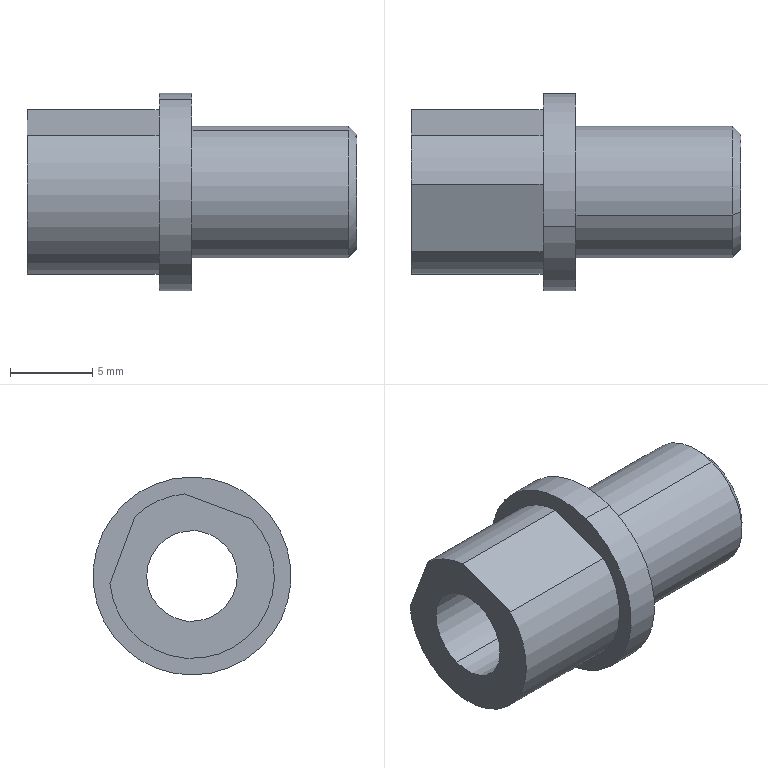Component | SolidWorks | 017NailOutlet-1 | 1 solid | 16 faces | box 20 x 12 x 12 mm | volume 856 mm3 | cylinder 8 | plane 6 | cone 2 | commonest cylinder face diameters 5.5 x2 8 x2 12 x2 10 x2
STEP:
#1=COLOUR_RGB('',0.7922,0.8196,0.9333);
#2=FILL_AREA_STYLE_COLOUR('',#1);
#3=FILL_AREA_STYLE('',(#2));
#4=SURFACE_STYLE_FILL_AREA(#3);
#5=SURFACE_SIDE_STYLE('',(#4));
#6=SURFACE_STYLE_USAGE(.BOTH.,#5);
#7=PRESENTATION_STYLE_ASSIGNMENT((#6));
#8=CARTESIAN_POINT('',(3.888,2.988,0.304));
#9=VERTEX_POINT('',#8);
#10=CARTESIAN_POINT('',(3.888,2.892,0.5621));
#11=VERTEX_POINT('',#10);
#12=CARTESIAN_POINT('',(3.888,2.94,0.4331));
#13=DIRECTION('',(1.,0.,0.));
#14=DIRECTION('',(0.,0.3505,-0.9366));
#15=AXIS2_PLACEMENT_3D('',#12,#13,#14);
#16=CIRCLE('',#15,0.1378);
#17=EDGE_CURVE('',#9,#11,#16,.T.);
#18=ORIENTED_EDGE('',*,*,#17,.F.);
#19=CARTESIAN_POINT('',(3.868,2.995,0.2856));
#20=VERTEX_POINT('',#19);
#21=CARTESIAN_POINT('',(3.888,2.988,0.304));
#22=DIRECTION('',(-0.7071,0.2478,-0.6623));
#23=VECTOR('',#22,39.37);
#24=LINE('',#21,#23);
#25=EDGE_CURVE('',#9,#20,#24,.T.);
#26=ORIENTED_EDGE('',*,*,#25,.T.);
#27=CARTESIAN_POINT('',(3.868,2.885,0.5806));
#28=VERTEX_POINT('',#27);
#29=CARTESIAN_POINT('',(3.868,2.94,0.4331));
#30=DIRECTION('',(-1.,-0.,-0.));
#31=DIRECTION('',(0.,0.3505,-0.9366));
#32=AXIS2_PLACEMENT_3D('',#29,#30,#31);
#33=CIRCLE('',#32,0.1575);
#34=EDGE_CURVE('',#28,#20,#33,.T.);
#35=ORIENTED_EDGE('',*,*,#34,.F.);
#36=CARTESIAN_POINT('',(3.888,2.892,0.5621));
#37=DIRECTION('',(-0.7071,-0.2478,0.6623));
#38=VECTOR('',#37,39.37);
#39=LINE('',#36,#38);
#40=EDGE_CURVE('',#11,#28,#39,.T.);
#41=ORIENTED_EDGE('',*,*,#40,.F.);
#42=EDGE_LOOP('',(#18,#26,#35,#41));
#43=FACE_OUTER_BOUND('',#42,.T.);
#44=CARTESIAN_POINT('',(3.888,2.94,0.4331));
#45=DIRECTION('',(-1.,-0.,-0.));
#46=DIRECTION('',(0.,-0.3505,0.9366));
#47=AXIS2_PLACEMENT_3D('',#44,#45,#46);
#48=CONICAL_SURFACE('',#47,0.1378,0.7854);
#49=ADVANCED_FACE('',(#43),#48,.T.);
#50=CARTESIAN_POINT('',(3.101,2.902,0.5345));
#51=VERTEX_POINT('',#50);
#52=CARTESIAN_POINT('',(3.101,2.978,0.3317));
#53=VERTEX_POINT('',#52);
#54=CARTESIAN_POINT('',(3.101,2.94,0.4331));
#55=DIRECTION('',(1.,0.,0.));
#56=DIRECTION('',(0.,0.3505,-0.9366));
#57=AXIS2_PLACEMENT_3D('',#54,#55,#56);
#58=CIRCLE('',#57,0.1083);
#59=EDGE_CURVE('',#51,#53,#58,.T.);
#60=ORIENTED_EDGE('',*,*,#59,.F.);
#61=CARTESIAN_POINT('',(3.888,2.902,0.5345));
#62=VERTEX_POINT('',#61);
#63=CARTESIAN_POINT('',(3.101,2.902,0.5345));
#64=DIRECTION('',(1.,0.,0.));
#65=VECTOR('',#64,39.37);
#66=LINE('',#63,#65);
#67=EDGE_CURVE('',#51,#62,#66,.T.);
#68=ORIENTED_EDGE('',*,*,#67,.T.);
#69=CARTESIAN_POINT('',(3.888,2.978,0.3317));
#70=VERTEX_POINT('',#69);
#71=CARTESIAN_POINT('',(3.888,2.94,0.4331));
#72=DIRECTION('',(1.,0.,0.));
#73=DIRECTION('',(0.,0.3505,-0.9366));
#74=AXIS2_PLACEMENT_3D('',#71,#72,#73);
#75=CIRCLE('',#74,0.1083);
#76=EDGE_CURVE('',#62,#70,#75,.T.);
#77=ORIENTED_EDGE('',*,*,#76,.T.);
#78=CARTESIAN_POINT('',(3.101,2.978,0.3317));
#79=DIRECTION('',(1.,0.,0.));
#80=VECTOR('',#79,39.37);
#81=LINE('',#78,#80);
#82=EDGE_CURVE('',#53,#70,#81,.T.);
#83=ORIENTED_EDGE('',*,*,#82,.F.);
#84=EDGE_LOOP('',(#60,#68,#77,#83));
#85=FACE_OUTER_BOUND('',#84,.T.);
#86=CARTESIAN_POINT('',(3.101,2.94,0.4331));
#87=DIRECTION('',(1.,0.,0.));
#88=DIRECTION('',(0.,0.3505,-0.9366));
#89=AXIS2_PLACEMENT_3D('',#86,#87,#88);
#90=CYLINDRICAL_SURFACE('',#89,0.1083);
#91=ADVANCED_FACE('',(#85),#90,.F.);
#92=ORIENTED_EDGE('',*,*,#34,.T.);
#93=CARTESIAN_POINT('',(3.494,2.995,0.2856));
#94=VERTEX_POINT('',#93);
#95=CARTESIAN_POINT('',(3.888,2.995,0.2856));
#96=DIRECTION('',(-1.,-0.,-0.));
#97=VECTOR('',#96,39.37);
#98=LINE('',#95,#97);
#99=EDGE_CURVE('',#20,#94,#98,.T.);
#100=ORIENTED_EDGE('',*,*,#99,.T.);
#101=CARTESIAN_POINT('',(3.494,2.885,0.5806));
#102=VERTEX_POINT('',#101);
#103=CARTESIAN_POINT('',(3.494,2.94,0.4331));
#104=DIRECTION('',(1.,0.,0.));
#105=DIRECTION('',(0.,0.3505,-0.9366));
#106=AXIS2_PLACEMENT_3D('',#103,#104,#105);
#107=CIRCLE('',#106,0.1575);
#108=EDGE_CURVE('',#94,#102,#107,.T.);
#109=ORIENTED_EDGE('',*,*,#108,.T.);
#110=CARTESIAN_POINT('',(3.888,2.885,0.5806));
#111=DIRECTION('',(-1.,-0.,-0.));
#112=VECTOR('',#111,39.37);
#113=LINE('',#110,#112);
#114=EDGE_CURVE('',#28,#102,#113,.T.);
#115=ORIENTED_EDGE('',*,*,#114,.F.);
#116=EDGE_LOOP('',(#92,#100,#109,#115));
#117=FACE_OUTER_BOUND('',#116,.T.);
#118=CARTESIAN_POINT('',(3.888,2.94,0.4331));
#119=DIRECTION('',(-1.,-0.,-0.));
#120=DIRECTION('',(0.,-0.3505,0.9366));
#121=AXIS2_PLACEMENT_3D('',#118,#119,#120);
#122=CYLINDRICAL_SURFACE('',#121,0.1575);
#123=ADVANCED_FACE('',(#117),#122,.T.);
#124=CARTESIAN_POINT('',(3.494,3.023,0.2118));
#125=VERTEX_POINT('',#124);
#126=CARTESIAN_POINT('',(3.494,2.857,0.6543));
#127=VERTEX_POINT('',#126);
#128=CARTESIAN_POINT('',(3.494,2.94,0.4331));
#129=DIRECTION('',(1.,0.,0.));
#130=DIRECTION('',(0.,0.3505,-0.9366));
#131=AXIS2_PLACEMENT_3D('',#128,#129,#130);
#132=CIRCLE('',#131,0.2362);
#133=EDGE_CURVE('',#125,#127,#132,.T.);
#134=ORIENTED_EDGE('',*,*,#133,.F.);
#135=CARTESIAN_POINT('',(3.416,3.023,0.2118));
#136=VERTEX_POINT('',#135);
#137=CARTESIAN_POINT('',(3.494,3.023,0.2118));
#138=DIRECTION('',(-1.,-0.,-0.));
#139=VECTOR('',#138,39.37);
#140=LINE('',#137,#139);
#141=EDGE_CURVE('',#125,#136,#140,.T.);
#142=ORIENTED_EDGE('',*,*,#141,.T.);
#143=CARTESIAN_POINT('',(3.416,2.857,0.6543));
#144=VERTEX_POINT('',#143);
#145=CARTESIAN_POINT('',(3.416,2.94,0.4331));
#146=DIRECTION('',(1.,0.,0.));
#147=DIRECTION('',(0.,0.3505,-0.9366));
#148=AXIS2_PLACEMENT_3D('',#145,#146,#147);
#149=CIRCLE('',#148,0.2362);
#150=EDGE_CURVE('',#136,#144,#149,.T.);
#151=ORIENTED_EDGE('',*,*,#150,.T.);
#152=CARTESIAN_POINT('',(3.494,2.857,0.6543));
#153=DIRECTION('',(-1.,-0.,-0.));
#154=VECTOR('',#153,39.37);
#155=LINE('',#152,#154);
#156=EDGE_CURVE('',#127,#144,#155,.T.);
#157=ORIENTED_EDGE('',*,*,#156,.F.);
#158=EDGE_LOOP('',(#134,#142,#151,#157));
#159=FACE_OUTER_BOUND('',#158,.T.);
#160=CARTESIAN_POINT('',(3.494,2.94,0.4331));
#161=DIRECTION('',(-1.,-0.,-0.));
#162=DIRECTION('',(0.,-0.3505,0.9366));
#163=AXIS2_PLACEMENT_3D('',#160,#161,#162);
#164=CYLINDRICAL_SURFACE('',#163,0.2362);
#165=ADVANCED_FACE('',(#159),#164,.T.);
#166=CARTESIAN_POINT('',(3.416,3.076,0.5755));
#167=VERTEX_POINT('',#166);
#168=CARTESIAN_POINT('',(3.416,2.958,0.6291));
#169=VERTEX_POINT('',#168);
#170=CARTESIAN_POINT('',(3.416,2.94,0.4331));
#171=DIRECTION('',(1.,0.,0.));
#172=DIRECTION('',(0.,0.3505,-0.9366));
#173=AXIS2_PLACEMENT_3D('',#170,#171,#172);
#174=CIRCLE('',#173,0.1969);
#175=EDGE_CURVE('',#167,#169,#174,.T.);
#176=ORIENTED_EDGE('',*,*,#175,.F.);
#177=CARTESIAN_POINT('',(3.101,3.076,0.5755));
#178=VERTEX_POINT('',#177);
#179=CARTESIAN_POINT('',(3.416,3.076,0.5755));
#180=DIRECTION('',(-1.,-0.,-0.));
#181=VECTOR('',#180,39.37);
#182=LINE('',#179,#181);
#183=EDGE_CURVE('',#167,#178,#182,.T.);
#184=ORIENTED_EDGE('',*,*,#183,.T.);
#185=CARTESIAN_POINT('',(3.101,2.958,0.6291));
#186=VERTEX_POINT('',#185);
#187=CARTESIAN_POINT('',(3.101,2.94,0.4331));
#188=DIRECTION('',(1.,0.,0.));
#189=DIRECTION('',(0.,0.3505,-0.9366));
#190=AXIS2_PLACEMENT_3D('',#187,#188,#189);
#191=CIRCLE('',#190,0.1969);
#192=EDGE_CURVE('',#178,#186,#191,.T.);
#193=ORIENTED_EDGE('',*,*,#192,.T.);
#194=CARTESIAN_POINT('',(3.416,2.958,0.6291));
#195=DIRECTION('',(-1.,-0.,-0.));
#196=VECTOR('',#195,39.37);
#197=LINE('',#194,#196);
#198=EDGE_CURVE('',#169,#186,#197,.T.);
#199=ORIENTED_EDGE('',*,*,#198,.F.);
#200=EDGE_LOOP('',(#176,#184,#193,#199));
#201=FACE_OUTER_BOUND('',#200,.T.);
#202=CARTESIAN_POINT('',(3.416,2.94,0.4331));
#203=DIRECTION('',(-1.,-0.,-0.));
#204=DIRECTION('',(0.,-0.3505,0.9366));
#205=AXIS2_PLACEMENT_3D('',#202,#203,#204);
#206=CYLINDRICAL_SURFACE('',#205,0.1969);
#207=ADVANCED_FACE('',(#201),#206,.T.);
#208=CARTESIAN_POINT('',(3.494,2.94,0.4331));
#209=DIRECTION('',(1.,0.,0.));
#210=DIRECTION('',(0.,0.3505,-0.9366));
#211=AXIS2_PLACEMENT_3D('',#208,#209,#210);
#212=CIRCLE('',#211,0.2362);
#213=EDGE_CURVE('',#127,#125,#212,.T.);
#214=ORIENTED_EDGE('',*,*,#213,.T.);
#215=ORIENTED_EDGE('',*,*,#133,.T.);
#216=EDGE_LOOP('',(#214,#215));
#217=FACE_OUTER_BOUND('',#216,.T.);
#218=CARTESIAN_POINT('',(3.494,2.94,0.4331));
#219=DIRECTION('',(1.,0.,0.));
#220=DIRECTION('',(0.,0.3505,-0.9366));
#221=AXIS2_PLACEMENT_3D('',#218,#219,#220);
#222=CIRCLE('',#221,0.1575);
#223=EDGE_CURVE('',#102,#94,#222,.T.);
#224=ORIENTED_EDGE('',*,*,#223,.F.);
#225=ORIENTED_EDGE('',*,*,#108,.F.);
#226=EDGE_LOOP('',(#224,#225));
#227=FACE_BOUND('',#226,.T.);
#228=CARTESIAN_POINT('',(3.494,2.94,0.4331));
#229=DIRECTION('',(1.,0.,0.));
#230=DIRECTION('',(-0.,0.3505,-0.9366));
#231=AXIS2_PLACEMENT_3D('',#228,#229,#230);
#232=PLANE('',#231);
#233=ADVANCED_FACE('',(#217,#227),#232,.T.);
#234=CARTESIAN_POINT('',(3.101,2.798,0.5689));
#235=VERTEX_POINT('',#234);
#236=CARTESIAN_POINT('',(3.101,3.136,0.4148));
#237=VERTEX_POINT('',#236);
#238=CARTESIAN_POINT('',(3.101,2.94,0.4331));
#239=DIRECTION('',(1.,0.,0.));
#240=DIRECTION('',(0.,0.3505,-0.9366));
#241=AXIS2_PLACEMENT_3D('',#238,#239,#240);
#242=CIRCLE('',#241,0.1969);
#243=EDGE_CURVE('',#235,#237,#242,.T.);
#244=ORIENTED_EDGE('',*,*,#243,.T.);
#245=CARTESIAN_POINT('',(3.416,3.136,0.4148));
#246=VERTEX_POINT('',#245);
#247=CARTESIAN_POINT('',(3.416,3.136,0.4148));
#248=DIRECTION('',(-1.,-0.,-0.));
#249=VECTOR('',#248,39.37);
#250=LINE('',#247,#249);
#251=EDGE_CURVE('',#246,#237,#250,.T.);
#252=ORIENTED_EDGE('',*,*,#251,.F.);
#253=CARTESIAN_POINT('',(3.416,2.798,0.5689));
#254=VERTEX_POINT('',#253);
#255=CARTESIAN_POINT('',(3.416,2.94,0.4331));
#256=DIRECTION('',(1.,0.,0.));
#257=DIRECTION('',(0.,0.3505,-0.9366));
#258=AXIS2_PLACEMENT_3D('',#255,#256,#257);
#259=CIRCLE('',#258,0.1969);
#260=EDGE_CURVE('',#254,#246,#259,.T.);
#261=ORIENTED_EDGE('',*,*,#260,.F.);
#262=CARTESIAN_POINT('',(3.416,2.798,0.5689));
#263=DIRECTION('',(-1.,-0.,-0.));
#264=VECTOR('',#263,39.37);
#265=LINE('',#262,#264);
#266=EDGE_CURVE('',#254,#235,#265,.T.);
#267=ORIENTED_EDGE('',*,*,#266,.T.);
#268=EDGE_LOOP('',(#244,#252,#261,#267));
#269=FACE_OUTER_BOUND('',#268,.T.);
#270=CARTESIAN_POINT('',(3.416,2.94,0.4331));
#271=DIRECTION('',(-1.,-0.,-0.));
#272=DIRECTION('',(0.,-0.3505,0.9366));
#273=AXIS2_PLACEMENT_3D('',#270,#271,#272);
#274=CYLINDRICAL_SURFACE('',#273,0.1969);
#275=ADVANCED_FACE('',(#269),#274,.T.);
#276=CARTESIAN_POINT('',(3.101,2.94,0.4331));
#277=DIRECTION('',(1.,0.,0.));
#278=DIRECTION('',(0.,0.3505,-0.9366));
#279=AXIS2_PLACEMENT_3D('',#276,#277,#278);
#280=CIRCLE('',#279,0.1083);
#281=EDGE_CURVE('',#53,#51,#280,.T.);
#282=ORIENTED_EDGE('',*,*,#281,.T.);
#283=ORIENTED_EDGE('',*,*,#59,.T.);
#284=EDGE_LOOP('',(#282,#283));
#285=FACE_BOUND('',#284,.T.);
#286=ORIENTED_EDGE('',*,*,#192,.F.);
#287=CARTESIAN_POINT('',(3.101,3.136,0.4148));
#288=DIRECTION('',(0.,-0.3505,0.9366));
#289=VECTOR('',#288,39.37);
#290=LINE('',#287,#289);
#291=EDGE_CURVE('',#237,#178,#290,.T.);
#292=ORIENTED_EDGE('',*,*,#291,.F.);
#293=ORIENTED_EDGE('',*,*,#243,.F.);
#294=CARTESIAN_POINT('',(3.101,2.958,0.6291));
#295=DIRECTION('',(0.,-0.9366,-0.3505));
#296=VECTOR('',#295,39.37);
#297=LINE('',#294,#296);
#298=EDGE_CURVE('',#186,#235,#297,.T.);
#299=ORIENTED_EDGE('',*,*,#298,.F.);
#300=EDGE_LOOP('',(#286,#292,#293,#299));
#301=FACE_OUTER_BOUND('',#300,.T.);
#302=CARTESIAN_POINT('',(3.101,2.94,0.4331));
#303=DIRECTION('',(1.,0.,0.));
#304=DIRECTION('',(-0.,0.3505,-0.9366));
#305=AXIS2_PLACEMENT_3D('',#302,#303,#304);
#306=PLANE('',#305);
#307=ADVANCED_FACE('',(#285,#301),#306,.F.);
#308=CARTESIAN_POINT('',(3.416,2.94,0.4331));
#309=DIRECTION('',(1.,0.,0.));
#310=DIRECTION('',(0.,0.3505,-0.9366));
#311=AXIS2_PLACEMENT_3D('',#308,#309,#310);
#312=CIRCLE('',#311,0.2362);
#313=EDGE_CURVE('',#144,#136,#312,.T.);
#314=ORIENTED_EDGE('',*,*,#313,.F.);
#315=ORIENTED_EDGE('',*,*,#150,.F.);
#316=EDGE_LOOP('',(#314,#315));
#317=FACE_OUTER_BOUND('',#316,.T.);
#318=ORIENTED_EDGE('',*,*,#260,.T.);
#319=CARTESIAN_POINT('',(3.416,3.136,0.4148));
#320=DIRECTION('',(0.,-0.3505,0.9366));
#321=VECTOR('',#320,39.37);
#322=LINE('',#319,#321);
#323=EDGE_CURVE('',#246,#167,#322,.T.);
#324=ORIENTED_EDGE('',*,*,#323,.T.);
#325=ORIENTED_EDGE('',*,*,#175,.T.);
#326=CARTESIAN_POINT('',(3.416,2.958,0.6291));
#327=DIRECTION('',(0.,-0.9366,-0.3505));
#328=VECTOR('',#327,39.37);
#329=LINE('',#326,#328);
#330=EDGE_CURVE('',#169,#254,#329,.T.);
#331=ORIENTED_EDGE('',*,*,#330,.T.);
#332=EDGE_LOOP('',(#318,#324,#325,#331));
#333=FACE_BOUND('',#332,.T.);
#334=CARTESIAN_POINT('',(3.416,2.94,0.4331));
#335=DIRECTION('',(1.,0.,0.));
#336=DIRECTION('',(-0.,0.3505,-0.9366));
#337=AXIS2_PLACEMENT_3D('',#334,#335,#336);
#338=PLANE('',#337);
#339=ADVANCED_FACE('',(#317,#333),#338,.F.);
#340=ORIENTED_EDGE('',*,*,#141,.F.);
#341=ORIENTED_EDGE('',*,*,#213,.F.);
#342=ORIENTED_EDGE('',*,*,#156,.T.);
#343=ORIENTED_EDGE('',*,*,#313,.T.);
#344=EDGE_LOOP('',(#340,#341,#342,#343));
#345=FACE_OUTER_BOUND('',#344,.T.);
#346=CARTESIAN_POINT('',(3.494,2.94,0.4331));
#347=DIRECTION('',(-1.,-0.,-0.));
#348=DIRECTION('',(0.,-0.3505,0.9366));
#349=AXIS2_PLACEMENT_3D('',#346,#347,#348);
#350=CYLINDRICAL_SURFACE('',#349,0.2362);
#351=ADVANCED_FACE('',(#345),#350,.T.);
#352=ORIENTED_EDGE('',*,*,#99,.F.);
#353=CARTESIAN_POINT('',(3.868,2.94,0.4331));
#354=DIRECTION('',(-1.,-0.,-0.));
#355=DIRECTION('',(0.,0.3505,-0.9366));
#356=AXIS2_PLACEMENT_3D('',#353,#354,#355);
#357=CIRCLE('',#356,0.1575);
#358=EDGE_CURVE('',#20,#28,#357,.T.);
#359=ORIENTED_EDGE('',*,*,#358,.T.);
#360=ORIENTED_EDGE('',*,*,#114,.T.);
#361=ORIENTED_EDGE('',*,*,#223,.T.);
#362=EDGE_LOOP('',(#352,#359,#360,#361));
#363=FACE_OUTER_BOUND('',#362,.T.);
#364=CARTESIAN_POINT('',(3.888,2.94,0.4331));
#365=DIRECTION('',(-1.,-0.,-0.));
#366=DIRECTION('',(0.,-0.3505,0.9366));
#367=AXIS2_PLACEMENT_3D('',#364,#365,#366);
#368=CYLINDRICAL_SURFACE('',#367,0.1575);
#369=ADVANCED_FACE('',(#363),#368,.T.);
#370=CARTESIAN_POINT('',(3.888,2.94,0.4331));
#371=DIRECTION('',(1.,0.,0.));
#372=DIRECTION('',(0.,0.3505,-0.9366));
#373=AXIS2_PLACEMENT_3D('',#370,#371,#372);
#374=CIRCLE('',#373,0.1378);
#375=EDGE_CURVE('',#11,#9,#374,.T.);
#376=ORIENTED_EDGE('',*,*,#375,.T.);
#377=ORIENTED_EDGE('',*,*,#17,.T.);
#378=EDGE_LOOP('',(#376,#377));
#379=FACE_OUTER_BOUND('',#378,.T.);
#380=CARTESIAN_POINT('',(3.888,2.94,0.4331));
#381=DIRECTION('',(1.,0.,0.));
#382=DIRECTION('',(0.,0.3505,-0.9366));
#383=AXIS2_PLACEMENT_3D('',#380,#381,#382);
#384=CIRCLE('',#383,0.1083);
#385=EDGE_CURVE('',#70,#62,#384,.T.);
#386=ORIENTED_EDGE('',*,*,#385,.F.);
#387=ORIENTED_EDGE('',*,*,#76,.F.);
#388=EDGE_LOOP('',(#386,#387));
#389=FACE_BOUND('',#388,.T.);
#390=CARTESIAN_POINT('',(3.888,2.94,0.4331));
#391=DIRECTION('',(1.,0.,0.));
#392=DIRECTION('',(-0.,0.3505,-0.9366));
#393=AXIS2_PLACEMENT_3D('',#390,#391,#392);
#394=PLANE('',#393);
#395=ADVANCED_FACE('',(#379,#389),#394,.T.);
#396=ORIENTED_EDGE('',*,*,#67,.F.);
#397=ORIENTED_EDGE('',*,*,#281,.F.);
#398=ORIENTED_EDGE('',*,*,#82,.T.);
#399=ORIENTED_EDGE('',*,*,#385,.T.);
#400=EDGE_LOOP('',(#396,#397,#398,#399));
#401=FACE_OUTER_BOUND('',#400,.T.);
#402=CARTESIAN_POINT('',(3.101,2.94,0.4331));
#403=DIRECTION('',(1.,0.,0.));
#404=DIRECTION('',(0.,0.3505,-0.9366));
#405=AXIS2_PLACEMENT_3D('',#402,#403,#404);
#406=CYLINDRICAL_SURFACE('',#405,0.1083);
#407=ADVANCED_FACE('',(#401),#406,.F.);
#408=ORIENTED_EDGE('',*,*,#25,.F.);
#409=ORIENTED_EDGE('',*,*,#375,.F.);
#410=ORIENTED_EDGE('',*,*,#40,.T.);
#411=ORIENTED_EDGE('',*,*,#358,.F.);
#412=EDGE_LOOP('',(#408,#409,#410,#411));
#413=FACE_OUTER_BOUND('',#412,.T.);
#414=CARTESIAN_POINT('',(3.888,2.94,0.4331));
#415=DIRECTION('',(-1.,-0.,-0.));
#416=DIRECTION('',(0.,-0.3505,0.9366));
#417=AXIS2_PLACEMENT_3D('',#414,#415,#416);
#418=CONICAL_SURFACE('',#417,0.1378,0.7854);
#419=ADVANCED_FACE('',(#413),#418,.T.);
#420=ORIENTED_EDGE('',*,*,#298,.T.);
#421=ORIENTED_EDGE('',*,*,#266,.F.);
#422=ORIENTED_EDGE('',*,*,#330,.F.);
#423=ORIENTED_EDGE('',*,*,#198,.T.);
#424=EDGE_LOOP('',(#420,#421,#422,#423));
#425=FACE_OUTER_BOUND('',#424,.T.);
#426=CARTESIAN_POINT('',(3.416,2.958,0.6291));
#427=DIRECTION('',(-0.,0.3505,-0.9366));
#428=DIRECTION('',(-1.,-0.,-0.));
#429=AXIS2_PLACEMENT_3D('',#426,#427,#428);
#430=PLANE('',#429);
#431=ADVANCED_FACE('',(#425),#430,.F.);
#432=ORIENTED_EDGE('',*,*,#291,.T.);
#433=ORIENTED_EDGE('',*,*,#183,.F.);
#434=ORIENTED_EDGE('',*,*,#323,.F.);
#435=ORIENTED_EDGE('',*,*,#251,.T.);
#436=EDGE_LOOP('',(#432,#433,#434,#435));
#437=FACE_OUTER_BOUND('',#436,.T.);
#438=CARTESIAN_POINT('',(3.416,3.136,0.4148));
#439=DIRECTION('',(0.,-0.9366,-0.3505));
#440=DIRECTION('',(-0.,0.3505,-0.9366));
#441=AXIS2_PLACEMENT_3D('',#438,#439,#440);
#442=PLANE('',#441);
#443=ADVANCED_FACE('',(#437),#442,.F.);
#444=CLOSED_SHELL('',(#49,#91,#123,#165,#207,#233,#275,#307,#339,#351,#369,#395,#407,#419,#431,#443));
#445=MANIFOLD_SOLID_BREP('',#444);
#446=STYLED_ITEM('',(#7),#445);
#447=PRESENTATION_LAYER_ASSIGNMENT('','',(#446));
#448=CARTESIAN_POINT('',(0.,0.,0.));
#449=DIRECTION('',(0.,0.,1.));
#450=DIRECTION('',(1.,0.,0.));
#451=AXIS2_PLACEMENT_3D('',#448,#449,#450);
#452=(LENGTH_UNIT()NAMED_UNIT(*)SI_UNIT($,.METRE.));
#453=LENGTH_MEASURE_WITH_UNIT(LENGTH_MEASURE(0.0254),#452);
#454=DIMENSIONAL_EXPONENTS(1.,0.,0.,0.,0.,0.,0.);
#455=(CONVERSION_BASED_UNIT('',#453)LENGTH_UNIT()NAMED_UNIT(#454));
#456=UNCERTAINTY_MEASURE_WITH_UNIT(LENGTH_MEASURE(0.00001),#455,'','');
#457=(NAMED_UNIT(*)PLANE_ANGLE_UNIT()SI_UNIT($,.RADIAN.));
#458=(NAMED_UNIT(*)SI_UNIT($,.STERADIAN.)SOLID_ANGLE_UNIT());
#459=(GEOMETRIC_REPRESENTATION_CONTEXT(3)GLOBAL_UNCERTAINTY_ASSIGNED_CONTEXT((#456))GLOBAL_UNIT_ASSIGNED_CONTEXT((#455,#457,#458))REPRESENTATION_CONTEXT('',''));
#460=ADVANCED_BREP_SHAPE_REPRESENTATION('',(#445,#451),#459);
#461=(LENGTH_UNIT()NAMED_UNIT(*)SI_UNIT($,.METRE.));
#462=LENGTH_MEASURE_WITH_UNIT(LENGTH_MEASURE(0.0254),#461);
#463=DIMENSIONAL_EXPONENTS(1.,0.,0.,0.,0.,0.,0.);
#464=(CONVERSION_BASED_UNIT('',#462)LENGTH_UNIT()NAMED_UNIT(#463));
#465=UNCERTAINTY_MEASURE_WITH_UNIT(LENGTH_MEASURE(0.00001),#464,'','');
#466=(NAMED_UNIT(*)PLANE_ANGLE_UNIT()SI_UNIT($,.RADIAN.));
#467=(NAMED_UNIT(*)SI_UNIT($,.STERADIAN.)SOLID_ANGLE_UNIT());
#468=(GEOMETRIC_REPRESENTATION_CONTEXT(3)GLOBAL_UNCERTAINTY_ASSIGNED_CONTEXT((#465))GLOBAL_UNIT_ASSIGNED_CONTEXT((#464,#466,#467))REPRESENTATION_CONTEXT('',''));
#469=MECHANICAL_DESIGN_GEOMETRIC_PRESENTATION_REPRESENTATION('',(#446),#468);